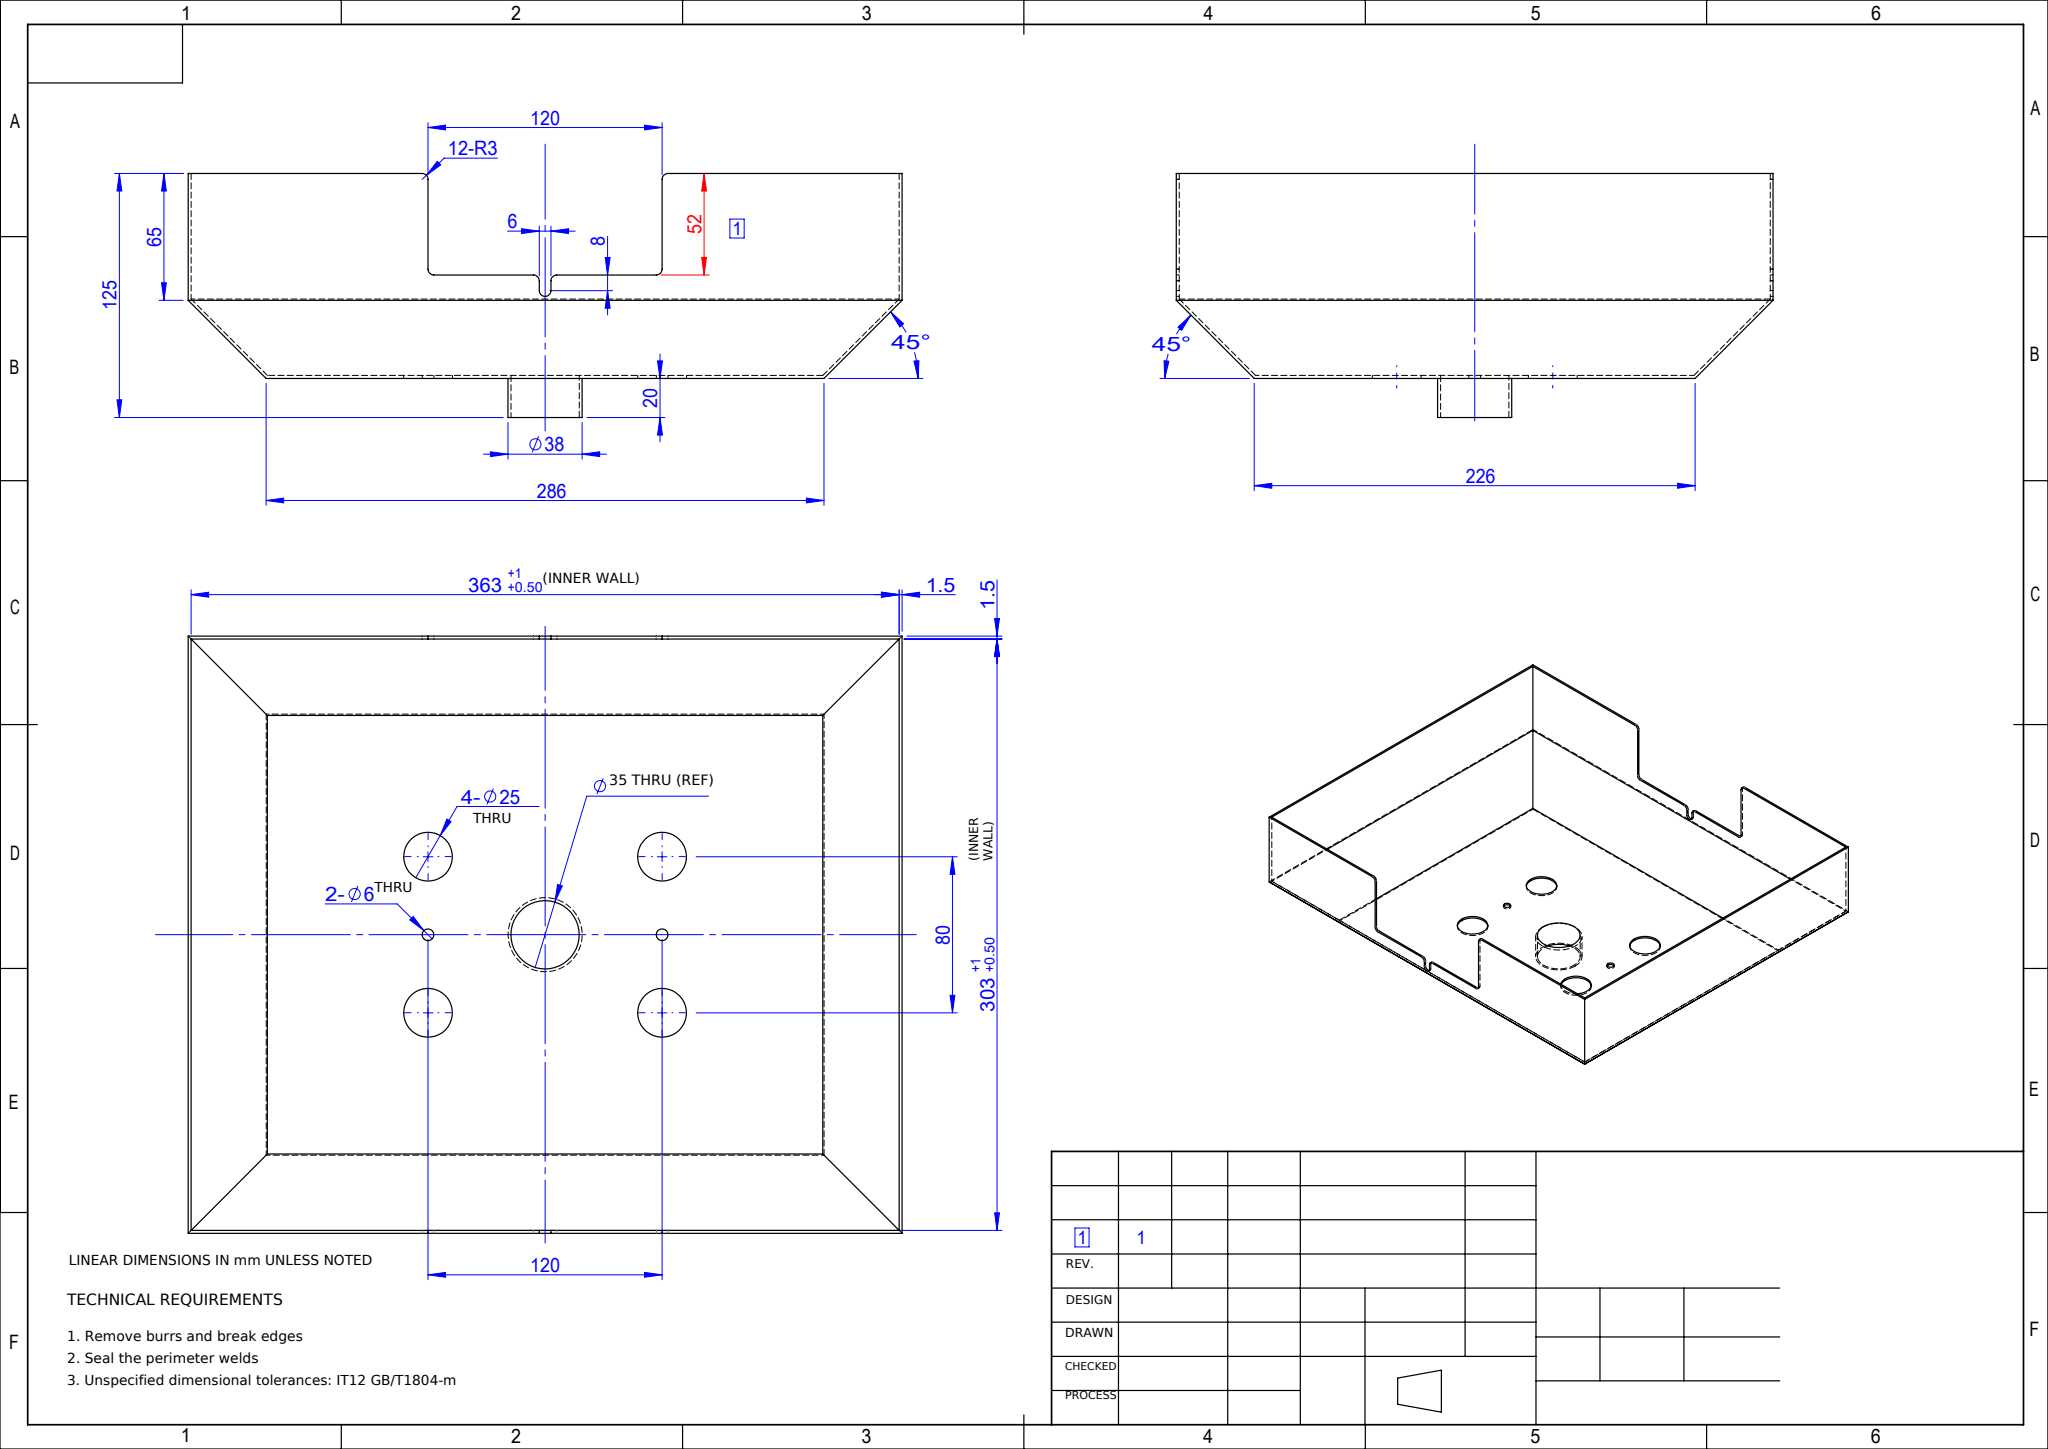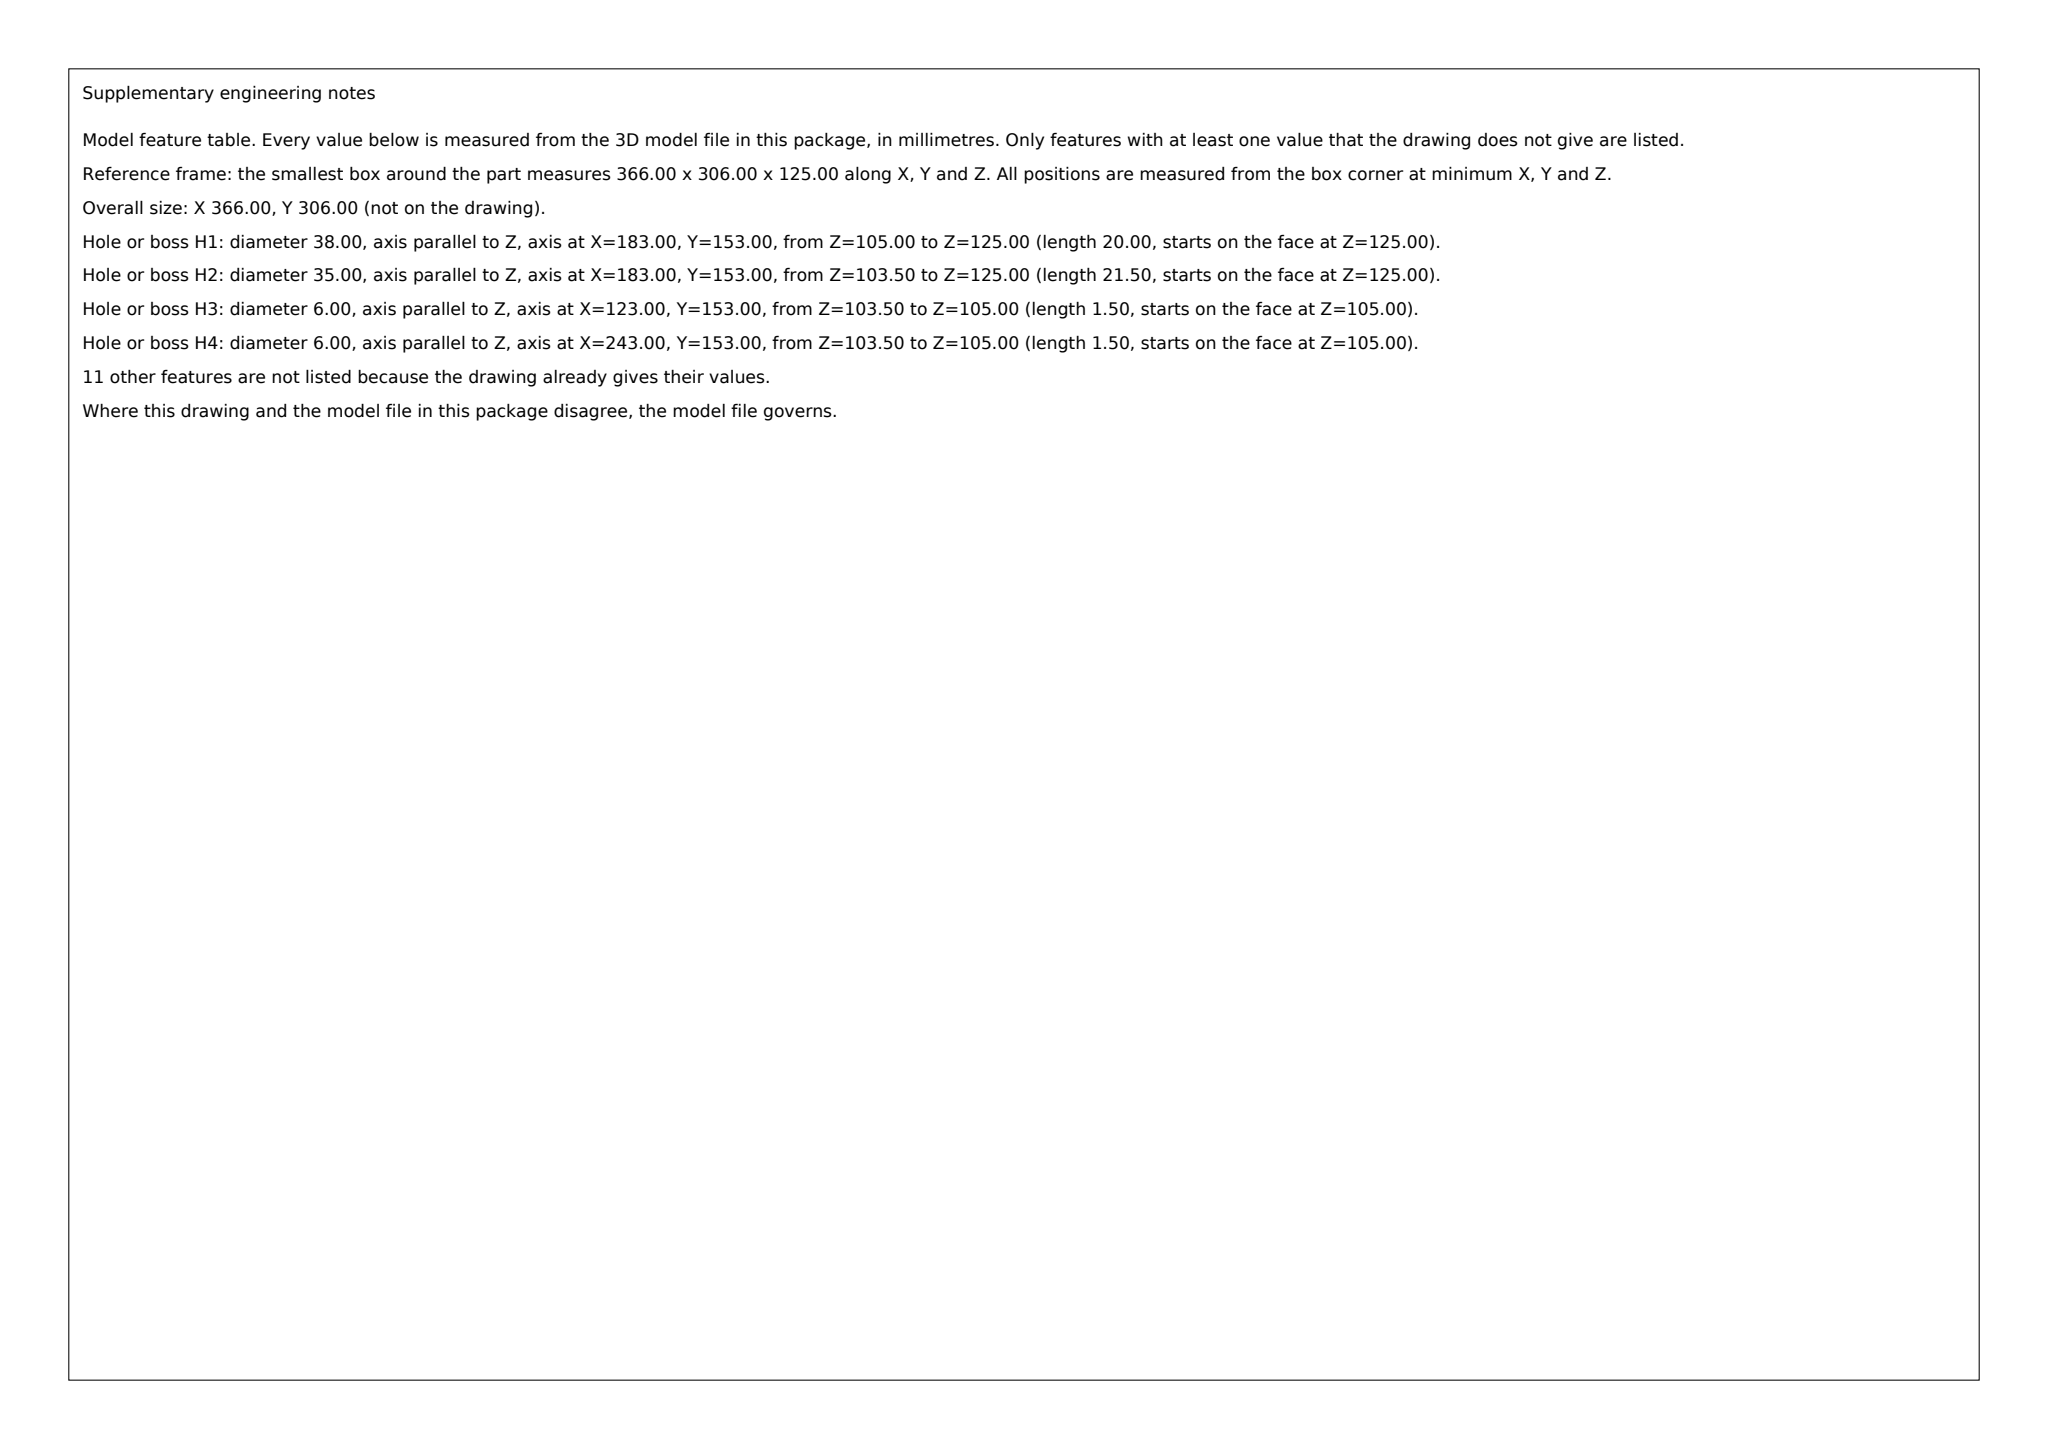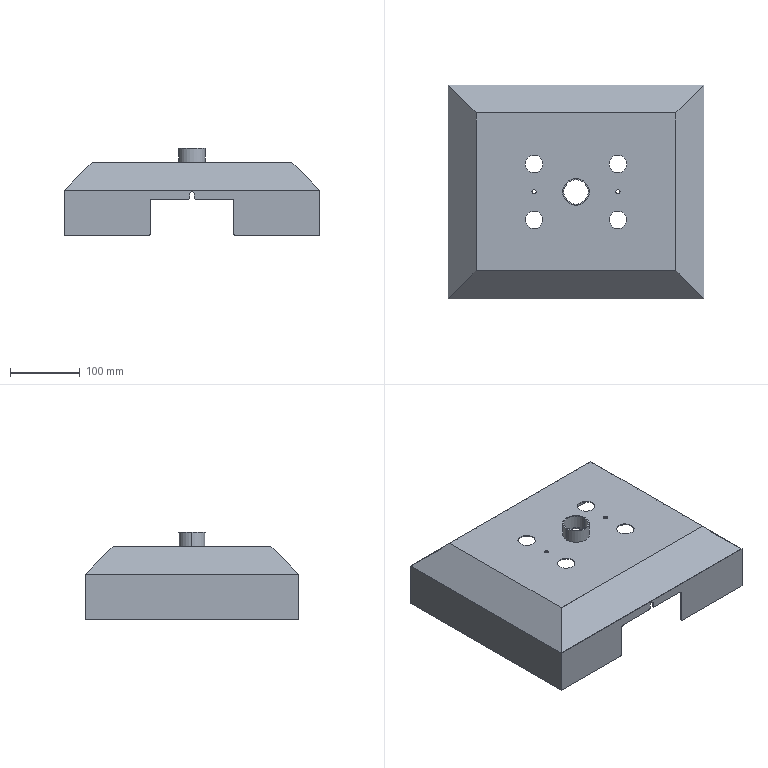Part | SolidWorks | mm | 1 solid | 65 faces | box 366 x 306 x 125 mm | volume 305366 mm3 | plane 33 | cylinder 32 | commonest cylinder face diameters 6 x20 25 x8 35 x2 38 x2
build123d program:
from build123d import *

# Parameters (mm, degrees)
SKETCH1_W                = 366
SKETCH1_H                = 306
BOSS_EXTRUDE1_DEPTH      = 40
BOSS_EXTRUDE1_TAPER      = 45
SKETCH2_W                = 366
SKETCH2_H                = 306
BOSS_EXTRUDE2_DEPTH      = 65
SKETCH3_R                = 19
BOSS_EXTRUDE3_DEPTH      = 20
SHELL1_T                 = -1.5
SKETCH5_R                = 12.5
CUT_EXTRUDE1_DEPTH       = 261.02
F_6_0_6_DIAMETER_HOLE3_D = 6
SKETCH16_W               = 120
SKETCH16_H               = 52
CUT_EXTRUDE3_DEPTH       = 363.422
FILLET1_R                = 3
CUT_EXTRUDE4_DEPTH       = 363.422
FILLET2_R                = 3


with BuildPart() as part:
    # Sketch1 → Boss-Extrude1 (new body)
    with BuildSketch(Plane.XY):
        Rectangle(SKETCH1_W, SKETCH1_H)
    extrude(amount=BOSS_EXTRUDE1_DEPTH, taper=BOSS_EXTRUDE1_TAPER)

    # Sketch2 → Boss-Extrude2 (add)
    with BuildSketch(Plane(origin=(0, 0, 0), x_dir=(-1, 0, 0), z_dir=(0, 0, -1))):
        Rectangle(SKETCH2_W, SKETCH2_H)
    extrude(amount=BOSS_EXTRUDE2_DEPTH)

    # Sketch3 → Boss-Extrude3 (add)
    with BuildSketch(Plane.XY.offset(40)):
        with Locations(Location((0, 0, 0), (0, 0, 180))):
            Circle(SKETCH3_R)
    extrude(amount=BOSS_EXTRUDE3_DEPTH)

    # Shell1
    shell1_openings = [part.faces().sort_by_distance(p)[0] for p in [
        (0, 0, -65),
        (0, 0, 60),
    ]]
    offset(amount=SHELL1_T, openings=shell1_openings, kind=Kind.INTERSECTION)

    # Sketch5 → Cut-Extrude1 (cut, through all)
    with BuildSketch(Plane(origin=(0, 0, 38.5), x_dir=(-1, 0, 0), z_dir=(0, 0, -1))):
        with Locations((-60, 40)):
            Circle(SKETCH5_R)
        with Locations((60, 40)):
            Circle(SKETCH5_R)
        with Locations((-60, -40)):
            Circle(SKETCH5_R)
        with Locations((60, -40)):
            Circle(SKETCH5_R)
    extrude(amount=-CUT_EXTRUDE1_DEPTH, mode=Mode.SUBTRACT)

    # 6.0 _6_ Diameter Hole3 (through all)
    with Locations(Plane(origin=(0, 0, 38.5), x_dir=(-1, 0, 0), z_dir=(0, 0, -1))):
        with Locations((-60, 0), (60, 0)):
            Hole(F_6_0_6_DIAMETER_HOLE3_D / 2)

    # Sketch16 → Cut-Extrude3 (cut, through all)
    with BuildSketch(Plane(origin=(0, 153, 0), x_dir=(1, 0, 0), z_dir=(0, 1, 0))):
        with Locations((0, 39)):
            Rectangle(SKETCH16_W, SKETCH16_H)
    extrude(amount=-CUT_EXTRUDE3_DEPTH, mode=Mode.SUBTRACT)

    # Fillet1
    fillet1_edges = [part.edges().sort_by_distance(p)[0] for p in [
        (60, -152.25, -65),
        (60, -152.25, -13),
        (-60, -152.25, -13),
        (-60, -152.25, -65),
        (60, 152.25, -65),
        (60, 152.25, -13),
        (-60, 152.25, -13),
        (-60, 152.25, -65),
    ]]
    fillet(fillet1_edges, radius=FILLET1_R)

    # Sketch17 → Cut-Extrude4 (cut, through all)
    with BuildSketch(Plane(origin=(0, 153, 0), x_dir=(1, 0, 0), z_dir=(0, 1, 0))):
        with BuildLine():
            Line((3, 13), (3, 5))
            ThreePointArc((3, 5), (0, 2), (-3, 5))
            Line((-3, 5), (-3, 13))
            ThreePointArc((-3, 13), (0, 16), (3, 13))
        make_face()
    extrude(amount=-CUT_EXTRUDE4_DEPTH, mode=Mode.SUBTRACT)

    # Fillet2
    fillet2_edges = [part.edges().sort_by_distance(p)[0] for p in [
        (3, -152.25, -13),
        (-3, -152.25, -13),
        (-3, 152.25, -13),
        (3, 152.25, -13),
    ]]
    fillet(fillet2_edges, radius=FILLET2_R)


solid = part.part